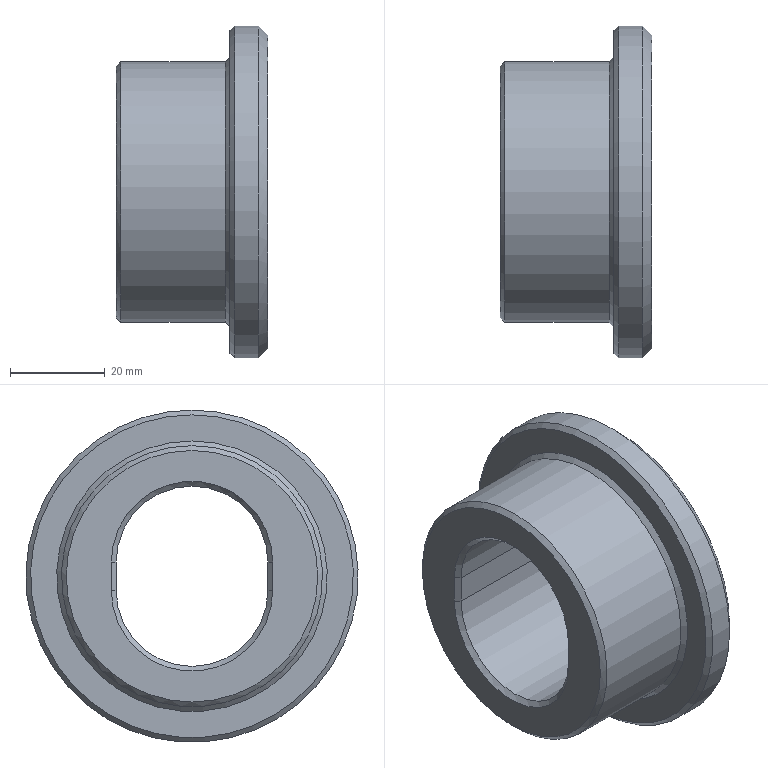CAM job | NX | mm | 3-axis | 1 set-up | 2 operations | part box 32 x 70 x 70
set-up 1
1. Adaptive Milling | Mill Mill5 12R0 | 1-D12 | path 5735.086 mm | 2.797 min
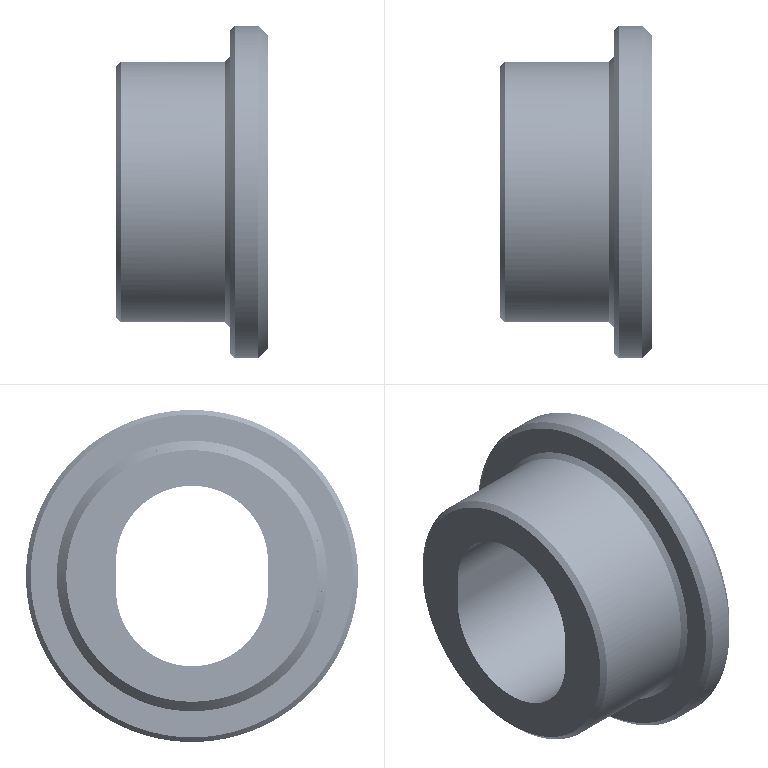2. Fixed-axis Surface Contouring | Mill Mill5 12R0 | 2-D12 | path 1207.377 mm | 0.5845 min